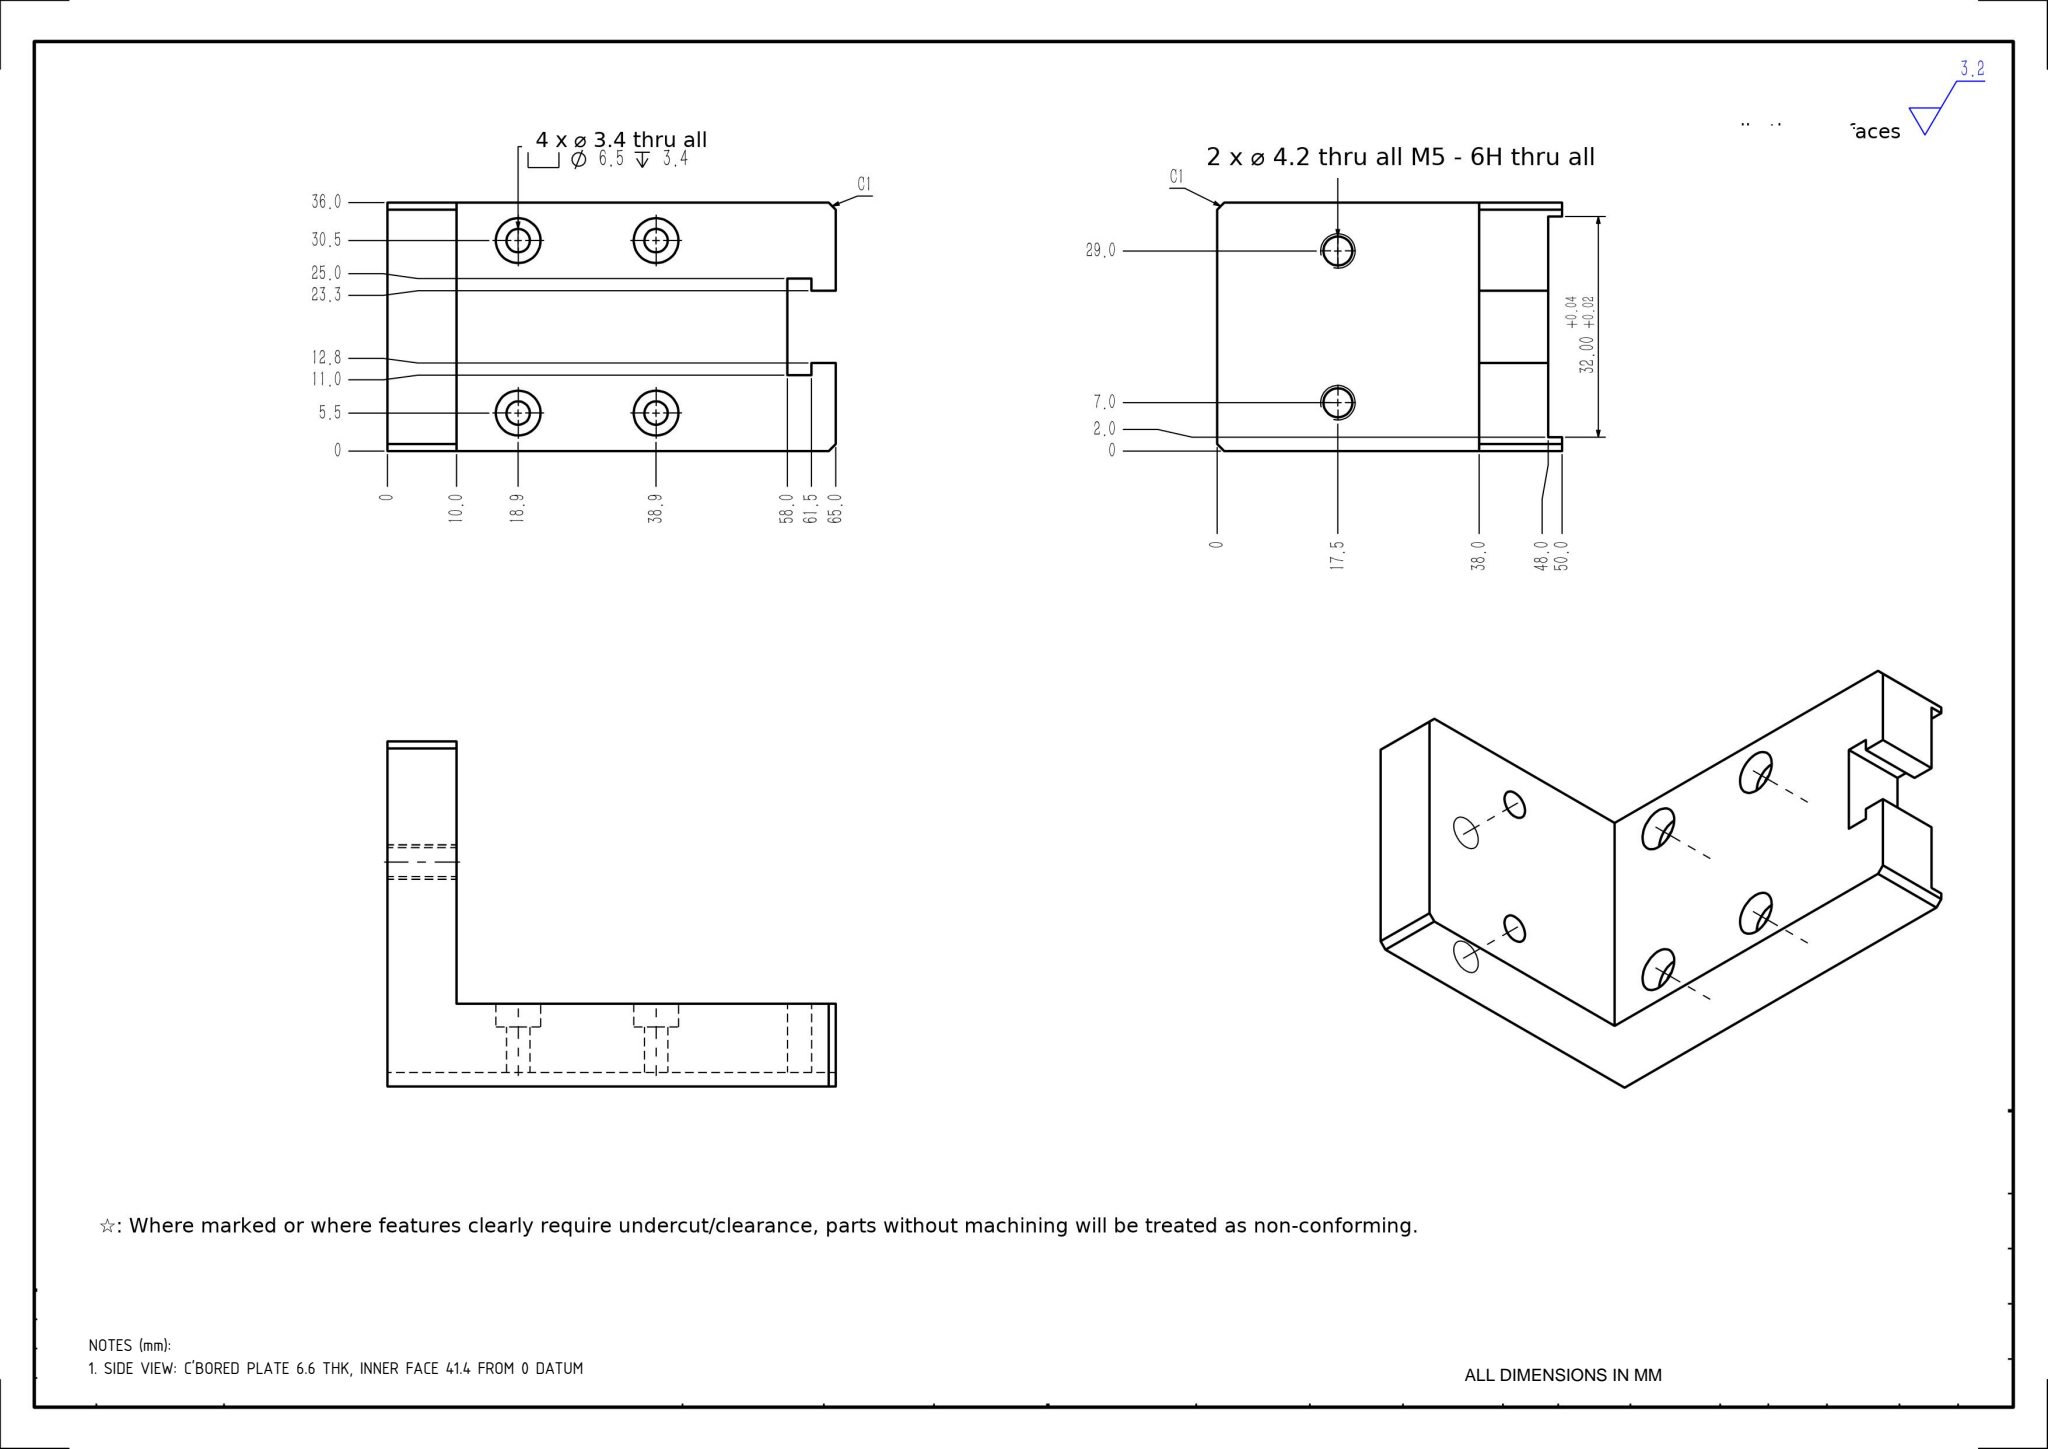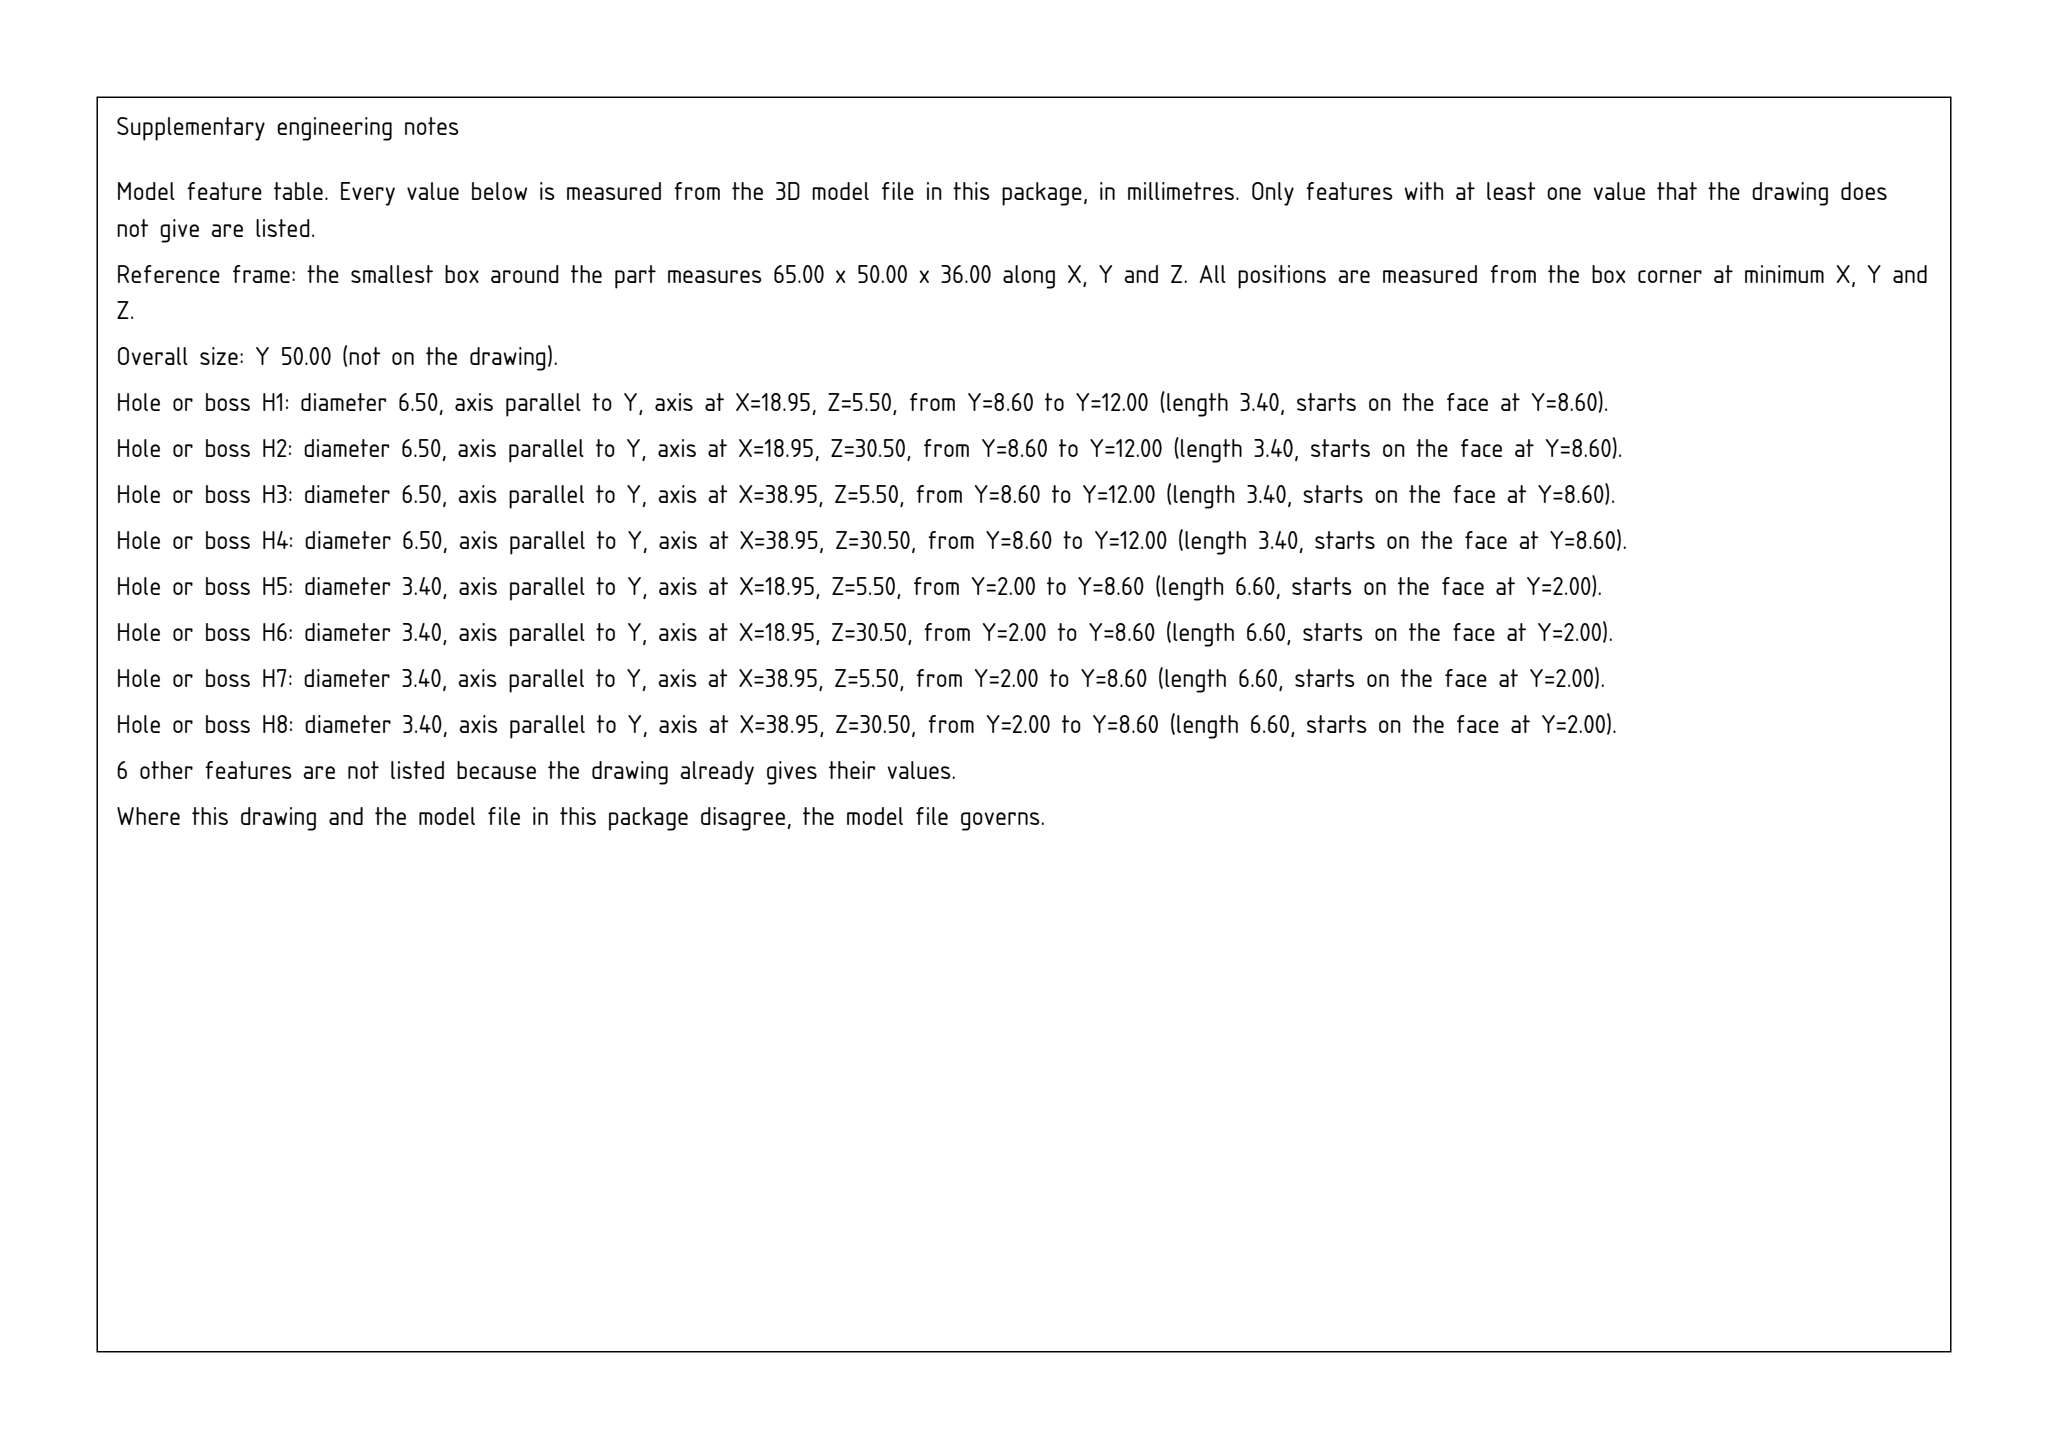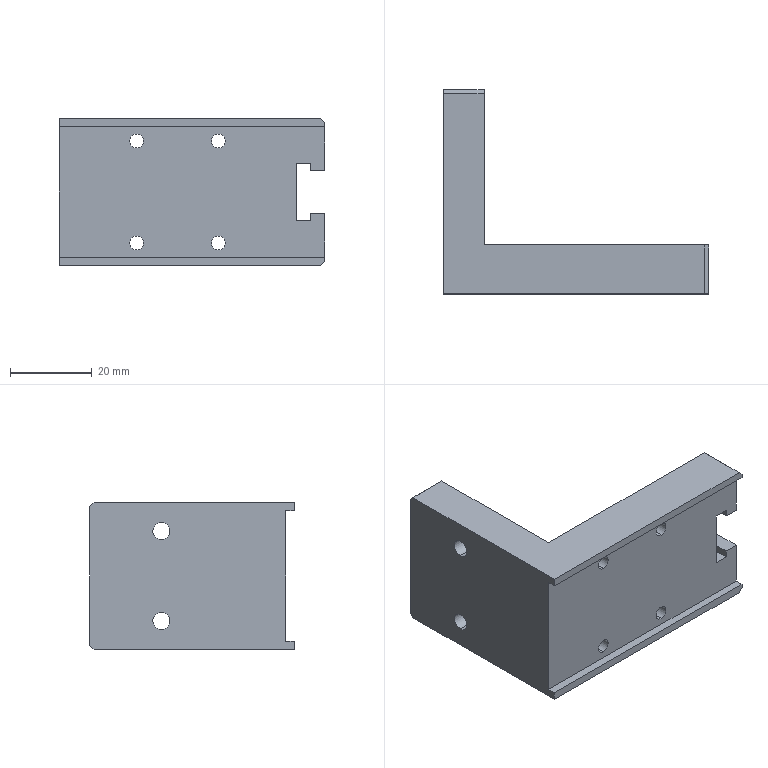Part | SolidWorks | mm | 1 solid | 48 faces | box 65 x 50 x 36 mm | volume 35752 mm3 | plane 28 | cylinder 20 | commonest cylinder face diameters 6.5 x8 3.4 x8 4.2 x4
Drawing notes:
SIDE VIEW: C'BORED PLATE 6.6 THK, INNER FACE 41.4 FROM 0 DATUM | from the solid: y-planes 2.0 and 8.6 (4 faces) => 6.6 thk; side-view datum y=50 => 50-8.6=41.4
build123d program:
from build123d import *

# Parameters (mm, degrees)
BOSS_EXTRUDE1_DEPTH                             = 18
SKETCH2_W                                       = 65
SKETCH2_H                                       = 32
CUT_EXTRUDE1_DEPTH                              = 2
CUT_EXTRUDE2_DEPTH                              = 54.144
M3_HEX_SOCKET_HEAD_CAP_SCREW_CBORE1_D           = 3.4
M3_HEX_SOCKET_HEAD_CAP_SCREW_CBORE1_CBORE_D     = 6.5
M3_HEX_SOCKET_HEAD_CAP_SCREW_CBORE1_CBORE_DEPTH = 3.4
M5_TAPPED_HOLE1_D                               = 4.2
CHAMFER1_SIZE                                   = 1


with BuildPart() as part:
    # Sketch1 → Boss-Extrude1 (new, symmetric)
    with BuildSketch(Plane.XY):
        Polygon((-22.5, 25), (-22.5, -13), (32.5, -13), (32.5, -25), (-32.5, -25), (-32.5, 25), align=None)
    extrude(amount=BOSS_EXTRUDE1_DEPTH, both=True)

    # Sketch2 → Cut-Extrude1 (cut)
    with BuildSketch(Plane(origin=(0, -25, 0), x_dir=(-1, 0, 0), z_dir=(0, -1, 0))):
        Rectangle(SKETCH2_W, SKETCH2_H)
    extrude(amount=-CUT_EXTRUDE1_DEPTH, mode=Mode.SUBTRACT)

    # Sketch3 → Cut-Extrude2 (cut, through all)
    with BuildSketch(Plane(origin=(0, -13, 0), x_dir=(1, 0, 0), z_dir=(0, 1, 0))):
        Polygon((29, -7), (25.5, -7), (25.5, 7), (29, 7), (29, 5.25), (32.5, 5.25), (32.5, -5.25), (29, -5.25), align=None)
    extrude(amount=-CUT_EXTRUDE2_DEPTH, mode=Mode.SUBTRACT)

    # M3 Hex Socket Head Cap Screw CBORE1 (through all)
    with Locations(Plane(origin=(0, -13, 0), x_dir=(1, 0, 0), z_dir=(0, 1, 0))):
        with Locations((-13.55, -12.5), (-13.55, 12.5), (6.45, -12.5), (6.45, 12.5)):
            CounterBoreHole(M3_HEX_SOCKET_HEAD_CAP_SCREW_CBORE1_D / 2, M3_HEX_SOCKET_HEAD_CAP_SCREW_CBORE1_CBORE_D / 2, M3_HEX_SOCKET_HEAD_CAP_SCREW_CBORE1_CBORE_DEPTH)

    # M5 Tapped Hole1 (through all)
    with Locations(Plane.ZY.offset(32.5)):
        with Locations((11, 7.5), (-11, 7.5)):
            Hole(M5_TAPPED_HOLE1_D / 2)

    # Chamfer1
    chamfer1_edges = [part.edges().sort_by_distance(p)[0] for p in [
        (32.5, -19, 18),
        (-27.5, 25, 18),
        (-27.5, 25, -18),
        (32.5, -19, -18),
    ]]
    chamfer(chamfer1_edges, length=CHAMFER1_SIZE)


solid = part.part